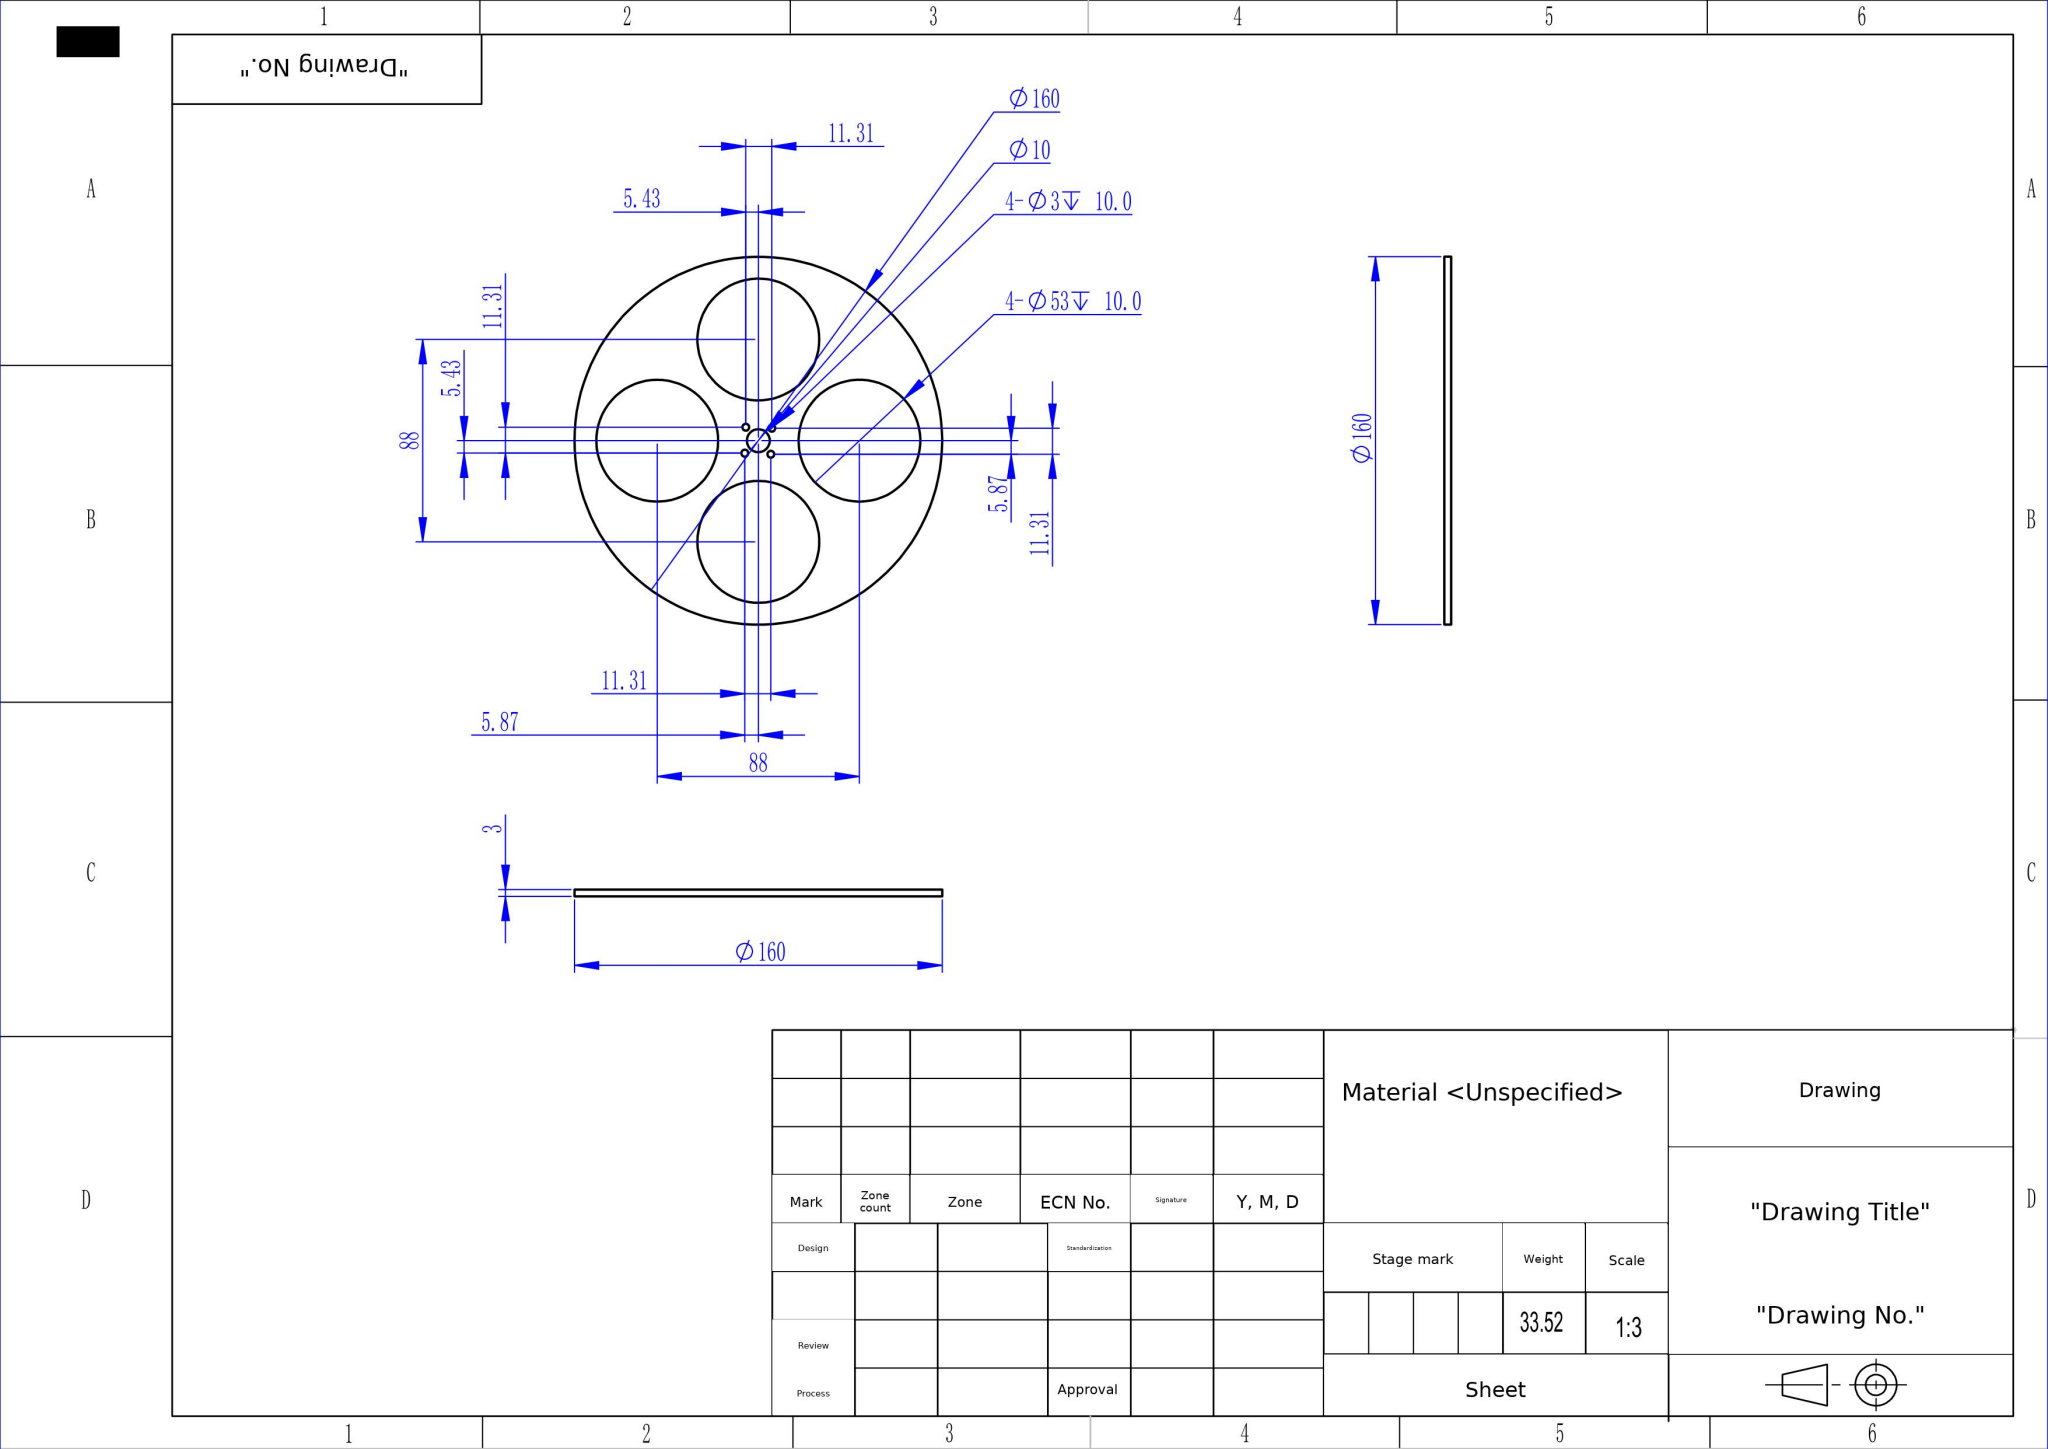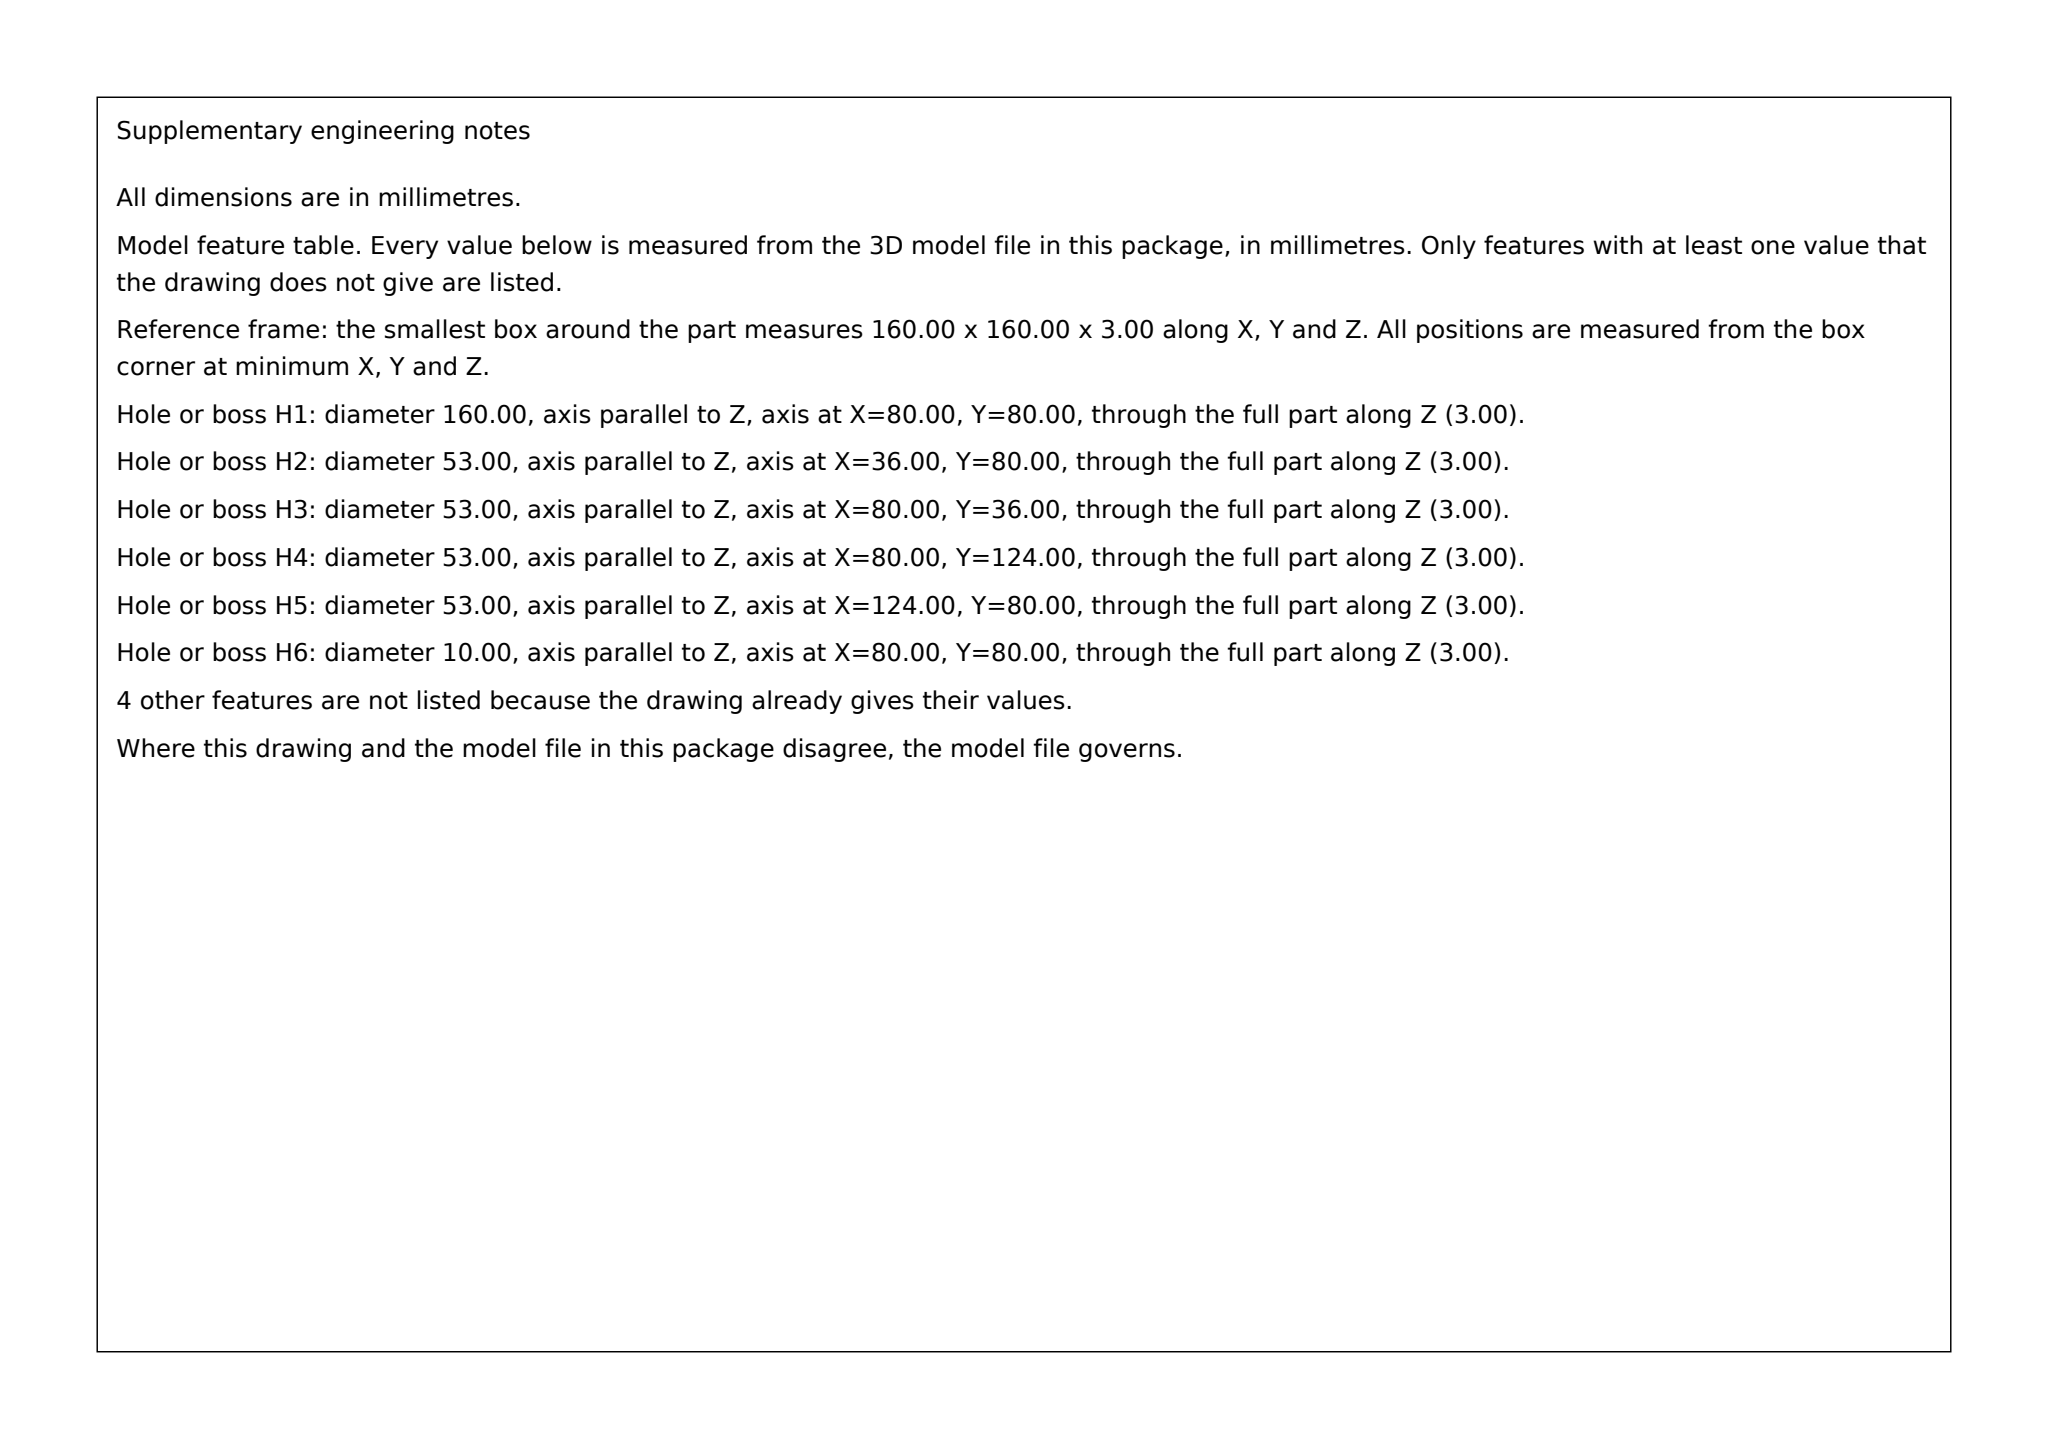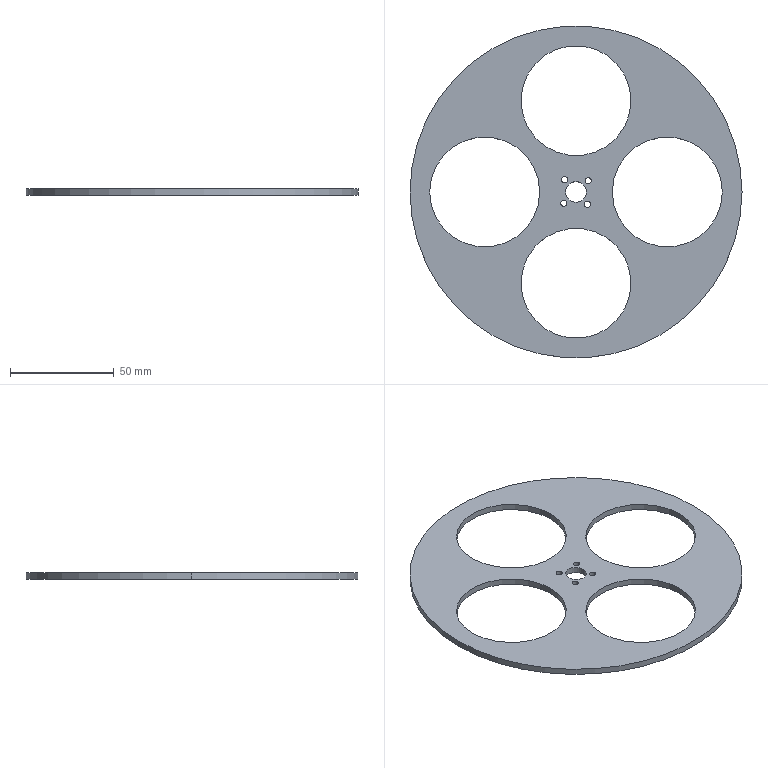Part | SolidWorks | mm | material <Unspecified> | 1 solid | 22 faces | box 160 x 160 x 3 mm | volume 33524 mm3 | cylinder 20 | plane 2 | commonest cylinder face diameters 3 x8 53 x8 10 x2 160 x2
build123d program:
from build123d import *

# Parameters (mm, degrees)
SKETCH1_R           = 80
SKETCH1_R_2         = 5
BOSS_EXTRUDE1_DEPTH = 3
SKETCH4_R           = 26.5
CUT_EXTRUDE2_DEPTH  = 10
CIRPATTERN1_COUNT   = 4
SKETCH5_R           = 1.5
CUT_EXTRUDE3_DEPTH  = 10


with BuildPart() as part:
    # Sketch1 → Boss-Extrude1 (new body)
    with BuildSketch(Plane.XY):
        Circle(SKETCH1_R)
        Circle(SKETCH1_R_2, mode=Mode.SUBTRACT)
    extrude(amount=BOSS_EXTRUDE1_DEPTH)

    # Sketch4 → Cut-Extrude2 (cut)
    with BuildSketch(Plane.XY.offset(3)):
        with Locations((0, 44)):
            Circle(SKETCH4_R)
    cut_extrude2 = extrude(amount=-CUT_EXTRUDE2_DEPTH, mode=Mode.SUBTRACT)

    # CirPattern1: Cut-Extrude2 ×4 about axis
    cirpattern1_axis = Axis((0, 0, 0), (0, 0, 1))
    for i in range(1, CIRPATTERN1_COUNT):
        add(cut_extrude2.rotate(cirpattern1_axis, i * 360 / CIRPATTERN1_COUNT), mode=Mode.SUBTRACT)

    # Sketch5 → Cut-Extrude3 (cut)
    with BuildSketch(Plane.XY.offset(3)):
        with Locations((-5.434, 5.871)):
            Circle(SKETCH5_R)
        with Locations((5.871, 5.434)):
            Circle(SKETCH5_R)
        with Locations((5.434, -5.871)):
            Circle(SKETCH5_R)
        with Locations((-5.871, -5.434)):
            Circle(SKETCH5_R)
    extrude(amount=-CUT_EXTRUDE3_DEPTH, mode=Mode.SUBTRACT)


solid = part.part
STEP:
#1=CARTESIAN_POINT('',(-7.371,-5.434,0.));
#2=VERTEX_POINT('',#1);
#3=CARTESIAN_POINT('',(-4.371,-5.434,0.));
#4=VERTEX_POINT('',#3);
#5=CARTESIAN_POINT('',(-5.871,-5.434,0.));
#6=DIRECTION('',(0.,0.,1.));
#7=DIRECTION('',(1.,0.,0.));
#8=AXIS2_PLACEMENT_3D('',#5,#6,#7);
#9=CIRCLE('',#8,1.5);
#10=EDGE_CURVE('',#2,#4,#9,.T.);
#11=ORIENTED_EDGE('',*,*,#10,.F.);
#12=CARTESIAN_POINT('',(-7.371,-5.434,3.));
#13=VERTEX_POINT('',#12);
#14=CARTESIAN_POINT('',(-7.371,-5.434,-7.));
#15=DIRECTION('',(0.,0.,1.));
#16=VECTOR('',#15,1000.);
#17=LINE('',#14,#16);
#18=EDGE_CURVE('',#2,#13,#17,.T.);
#19=ORIENTED_EDGE('',*,*,#18,.T.);
#20=CARTESIAN_POINT('',(-4.371,-5.434,3.));
#21=VERTEX_POINT('',#20);
#22=CARTESIAN_POINT('',(-5.871,-5.434,3.));
#23=DIRECTION('',(0.,0.,1.));
#24=DIRECTION('',(1.,0.,0.));
#25=AXIS2_PLACEMENT_3D('',#22,#23,#24);
#26=CIRCLE('',#25,1.5);
#27=EDGE_CURVE('',#13,#21,#26,.T.);
#28=ORIENTED_EDGE('',*,*,#27,.T.);
#29=CARTESIAN_POINT('',(-4.371,-5.434,-7.));
#30=DIRECTION('',(0.,0.,1.));
#31=VECTOR('',#30,1000.);
#32=LINE('',#29,#31);
#33=EDGE_CURVE('',#4,#21,#32,.T.);
#34=ORIENTED_EDGE('',*,*,#33,.F.);
#35=EDGE_LOOP('',(#11,#19,#28,#34));
#36=FACE_OUTER_BOUND('',#35,.T.);
#37=CARTESIAN_POINT('',(-5.871,-5.434,-7.));
#38=DIRECTION('',(0.,0.,1.));
#39=DIRECTION('',(1.,0.,0.));
#40=AXIS2_PLACEMENT_3D('',#37,#38,#39);
#41=CYLINDRICAL_SURFACE('',#40,1.5);
#42=ADVANCED_FACE('',(#36),#41,.F.);
#43=CARTESIAN_POINT('',(3.934,-5.871,0.));
#44=VERTEX_POINT('',#43);
#45=CARTESIAN_POINT('',(6.934,-5.871,0.));
#46=VERTEX_POINT('',#45);
#47=CARTESIAN_POINT('',(5.434,-5.871,0.));
#48=DIRECTION('',(0.,0.,1.));
#49=DIRECTION('',(1.,0.,0.));
#50=AXIS2_PLACEMENT_3D('',#47,#48,#49);
#51=CIRCLE('',#50,1.5);
#52=EDGE_CURVE('',#44,#46,#51,.T.);
#53=ORIENTED_EDGE('',*,*,#52,.F.);
#54=CARTESIAN_POINT('',(3.934,-5.871,3.));
#55=VERTEX_POINT('',#54);
#56=CARTESIAN_POINT('',(3.934,-5.871,-7.));
#57=DIRECTION('',(0.,0.,1.));
#58=VECTOR('',#57,1000.);
#59=LINE('',#56,#58);
#60=EDGE_CURVE('',#44,#55,#59,.T.);
#61=ORIENTED_EDGE('',*,*,#60,.T.);
#62=CARTESIAN_POINT('',(6.934,-5.871,3.));
#63=VERTEX_POINT('',#62);
#64=CARTESIAN_POINT('',(5.434,-5.871,3.));
#65=DIRECTION('',(0.,0.,1.));
#66=DIRECTION('',(1.,0.,0.));
#67=AXIS2_PLACEMENT_3D('',#64,#65,#66);
#68=CIRCLE('',#67,1.5);
#69=EDGE_CURVE('',#55,#63,#68,.T.);
#70=ORIENTED_EDGE('',*,*,#69,.T.);
#71=CARTESIAN_POINT('',(6.934,-5.871,-7.));
#72=DIRECTION('',(0.,0.,1.));
#73=VECTOR('',#72,1000.);
#74=LINE('',#71,#73);
#75=EDGE_CURVE('',#46,#63,#74,.T.);
#76=ORIENTED_EDGE('',*,*,#75,.F.);
#77=EDGE_LOOP('',(#53,#61,#70,#76));
#78=FACE_OUTER_BOUND('',#77,.T.);
#79=CARTESIAN_POINT('',(5.434,-5.871,-7.));
#80=DIRECTION('',(0.,0.,1.));
#81=DIRECTION('',(1.,0.,0.));
#82=AXIS2_PLACEMENT_3D('',#79,#80,#81);
#83=CYLINDRICAL_SURFACE('',#82,1.5);
#84=ADVANCED_FACE('',(#78),#83,.F.);
#85=CARTESIAN_POINT('',(4.371,5.434,0.));
#86=VERTEX_POINT('',#85);
#87=CARTESIAN_POINT('',(7.371,5.434,0.));
#88=VERTEX_POINT('',#87);
#89=CARTESIAN_POINT('',(5.871,5.434,0.));
#90=DIRECTION('',(0.,0.,1.));
#91=DIRECTION('',(1.,0.,0.));
#92=AXIS2_PLACEMENT_3D('',#89,#90,#91);
#93=CIRCLE('',#92,1.5);
#94=EDGE_CURVE('',#86,#88,#93,.T.);
#95=ORIENTED_EDGE('',*,*,#94,.F.);
#96=CARTESIAN_POINT('',(4.371,5.434,3.));
#97=VERTEX_POINT('',#96);
#98=CARTESIAN_POINT('',(4.371,5.434,-7.));
#99=DIRECTION('',(0.,0.,1.));
#100=VECTOR('',#99,1000.);
#101=LINE('',#98,#100);
#102=EDGE_CURVE('',#86,#97,#101,.T.);
#103=ORIENTED_EDGE('',*,*,#102,.T.);
#104=CARTESIAN_POINT('',(7.371,5.434,3.));
#105=VERTEX_POINT('',#104);
#106=CARTESIAN_POINT('',(5.871,5.434,3.));
#107=DIRECTION('',(0.,0.,1.));
#108=DIRECTION('',(1.,0.,0.));
#109=AXIS2_PLACEMENT_3D('',#106,#107,#108);
#110=CIRCLE('',#109,1.5);
#111=EDGE_CURVE('',#97,#105,#110,.T.);
#112=ORIENTED_EDGE('',*,*,#111,.T.);
#113=CARTESIAN_POINT('',(7.371,5.434,-7.));
#114=DIRECTION('',(0.,0.,1.));
#115=VECTOR('',#114,1000.);
#116=LINE('',#113,#115);
#117=EDGE_CURVE('',#88,#105,#116,.T.);
#118=ORIENTED_EDGE('',*,*,#117,.F.);
#119=EDGE_LOOP('',(#95,#103,#112,#118));
#120=FACE_OUTER_BOUND('',#119,.T.);
#121=CARTESIAN_POINT('',(5.871,5.434,-7.));
#122=DIRECTION('',(0.,0.,1.));
#123=DIRECTION('',(1.,0.,0.));
#124=AXIS2_PLACEMENT_3D('',#121,#122,#123);
#125=CYLINDRICAL_SURFACE('',#124,1.5);
#126=ADVANCED_FACE('',(#120),#125,.F.);
#127=CARTESIAN_POINT('',(-6.934,5.871,0.));
#128=VERTEX_POINT('',#127);
#129=CARTESIAN_POINT('',(-3.934,5.871,0.));
#130=VERTEX_POINT('',#129);
#131=CARTESIAN_POINT('',(-5.434,5.871,0.));
#132=DIRECTION('',(0.,0.,1.));
#133=DIRECTION('',(1.,0.,0.));
#134=AXIS2_PLACEMENT_3D('',#131,#132,#133);
#135=CIRCLE('',#134,1.5);
#136=EDGE_CURVE('',#128,#130,#135,.T.);
#137=ORIENTED_EDGE('',*,*,#136,.F.);
#138=CARTESIAN_POINT('',(-6.934,5.871,3.));
#139=VERTEX_POINT('',#138);
#140=CARTESIAN_POINT('',(-6.934,5.871,-7.));
#141=DIRECTION('',(0.,0.,1.));
#142=VECTOR('',#141,1000.);
#143=LINE('',#140,#142);
#144=EDGE_CURVE('',#128,#139,#143,.T.);
#145=ORIENTED_EDGE('',*,*,#144,.T.);
#146=CARTESIAN_POINT('',(-3.934,5.871,3.));
#147=VERTEX_POINT('',#146);
#148=CARTESIAN_POINT('',(-5.434,5.871,3.));
#149=DIRECTION('',(0.,0.,1.));
#150=DIRECTION('',(1.,0.,0.));
#151=AXIS2_PLACEMENT_3D('',#148,#149,#150);
#152=CIRCLE('',#151,1.5);
#153=EDGE_CURVE('',#139,#147,#152,.T.);
#154=ORIENTED_EDGE('',*,*,#153,.T.);
#155=CARTESIAN_POINT('',(-3.934,5.871,-7.));
#156=DIRECTION('',(0.,0.,1.));
#157=VECTOR('',#156,1000.);
#158=LINE('',#155,#157);
#159=EDGE_CURVE('',#130,#147,#158,.T.);
#160=ORIENTED_EDGE('',*,*,#159,.F.);
#161=EDGE_LOOP('',(#137,#145,#154,#160));
#162=FACE_OUTER_BOUND('',#161,.T.);
#163=CARTESIAN_POINT('',(-5.434,5.871,-7.));
#164=DIRECTION('',(0.,0.,1.));
#165=DIRECTION('',(1.,0.,0.));
#166=AXIS2_PLACEMENT_3D('',#163,#164,#165);
#167=CYLINDRICAL_SURFACE('',#166,1.5);
#168=ADVANCED_FACE('',(#162),#167,.F.);
#169=CARTESIAN_POINT('',(-26.5,-44.,0.));
#170=VERTEX_POINT('',#169);
#171=CARTESIAN_POINT('',(26.5,-44.,0.));
#172=VERTEX_POINT('',#171);
#173=CARTESIAN_POINT('',(0.,-44.,0.));
#174=DIRECTION('',(0.,0.,1.));
#175=DIRECTION('',(1.,0.,0.));
#176=AXIS2_PLACEMENT_3D('',#173,#174,#175);
#177=CIRCLE('',#176,26.5);
#178=EDGE_CURVE('',#170,#172,#177,.T.);
#179=ORIENTED_EDGE('',*,*,#178,.F.);
#180=CARTESIAN_POINT('',(-26.5,-44.,3.));
#181=VERTEX_POINT('',#180);
#182=CARTESIAN_POINT('',(-26.5,-44.,-7.));
#183=DIRECTION('',(0.,0.,1.));
#184=VECTOR('',#183,1000.);
#185=LINE('',#182,#184);
#186=EDGE_CURVE('',#170,#181,#185,.T.);
#187=ORIENTED_EDGE('',*,*,#186,.T.);
#188=CARTESIAN_POINT('',(26.5,-44.,3.));
#189=VERTEX_POINT('',#188);
#190=CARTESIAN_POINT('',(0.,-44.,3.));
#191=DIRECTION('',(0.,0.,1.));
#192=DIRECTION('',(-1.,0.,0.));
#193=AXIS2_PLACEMENT_3D('',#190,#191,#192);
#194=CIRCLE('',#193,26.5);
#195=EDGE_CURVE('',#181,#189,#194,.T.);
#196=ORIENTED_EDGE('',*,*,#195,.T.);
#197=CARTESIAN_POINT('',(26.5,-44.,-7.));
#198=DIRECTION('',(0.,0.,1.));
#199=VECTOR('',#198,1000.);
#200=LINE('',#197,#199);
#201=EDGE_CURVE('',#172,#189,#200,.T.);
#202=ORIENTED_EDGE('',*,*,#201,.F.);
#203=EDGE_LOOP('',(#179,#187,#196,#202));
#204=FACE_OUTER_BOUND('',#203,.T.);
#205=CARTESIAN_POINT('',(0.,-44.,-7.));
#206=DIRECTION('',(0.,0.,1.));
#207=DIRECTION('',(1.,0.,0.));
#208=AXIS2_PLACEMENT_3D('',#205,#206,#207);
#209=CYLINDRICAL_SURFACE('',#208,26.5);
#210=ADVANCED_FACE('',(#204),#209,.F.);
#211=CARTESIAN_POINT('',(17.5,0.,0.));
#212=VERTEX_POINT('',#211);
#213=CARTESIAN_POINT('',(70.5,0.,0.));
#214=VERTEX_POINT('',#213);
#215=CARTESIAN_POINT('',(44.,0.,0.));
#216=DIRECTION('',(0.,0.,1.));
#217=DIRECTION('',(1.,0.,0.));
#218=AXIS2_PLACEMENT_3D('',#215,#216,#217);
#219=CIRCLE('',#218,26.5);
#220=EDGE_CURVE('',#212,#214,#219,.T.);
#221=ORIENTED_EDGE('',*,*,#220,.F.);
#222=CARTESIAN_POINT('',(17.5,0.,3.));
#223=VERTEX_POINT('',#222);
#224=CARTESIAN_POINT('',(17.5,0.,-7.));
#225=DIRECTION('',(0.,0.,1.));
#226=VECTOR('',#225,1000.);
#227=LINE('',#224,#226);
#228=EDGE_CURVE('',#212,#223,#227,.T.);
#229=ORIENTED_EDGE('',*,*,#228,.T.);
#230=CARTESIAN_POINT('',(70.5,0.,3.));
#231=VERTEX_POINT('',#230);
#232=CARTESIAN_POINT('',(44.,0.,3.));
#233=DIRECTION('',(0.,0.,1.));
#234=DIRECTION('',(0.,-1.,0.));
#235=AXIS2_PLACEMENT_3D('',#232,#233,#234);
#236=CIRCLE('',#235,26.5);
#237=EDGE_CURVE('',#223,#231,#236,.T.);
#238=ORIENTED_EDGE('',*,*,#237,.T.);
#239=CARTESIAN_POINT('',(70.5,0.,-7.));
#240=DIRECTION('',(0.,0.,1.));
#241=VECTOR('',#240,1000.);
#242=LINE('',#239,#241);
#243=EDGE_CURVE('',#214,#231,#242,.T.);
#244=ORIENTED_EDGE('',*,*,#243,.F.);
#245=EDGE_LOOP('',(#221,#229,#238,#244));
#246=FACE_OUTER_BOUND('',#245,.T.);
#247=CARTESIAN_POINT('',(44.,0.,-7.));
#248=DIRECTION('',(0.,0.,1.));
#249=DIRECTION('',(1.,0.,0.));
#250=AXIS2_PLACEMENT_3D('',#247,#248,#249);
#251=CYLINDRICAL_SURFACE('',#250,26.5);
#252=ADVANCED_FACE('',(#246),#251,.F.);
#253=CARTESIAN_POINT('',(-70.5,-0.,0.));
#254=VERTEX_POINT('',#253);
#255=CARTESIAN_POINT('',(-17.5,-0.,0.));
#256=VERTEX_POINT('',#255);
#257=CARTESIAN_POINT('',(-44.,-0.,0.));
#258=DIRECTION('',(0.,0.,1.));
#259=DIRECTION('',(1.,0.,0.));
#260=AXIS2_PLACEMENT_3D('',#257,#258,#259);
#261=CIRCLE('',#260,26.5);
#262=EDGE_CURVE('',#254,#256,#261,.T.);
#263=ORIENTED_EDGE('',*,*,#262,.F.);
#264=CARTESIAN_POINT('',(-70.5,-0.,3.));
#265=VERTEX_POINT('',#264);
#266=CARTESIAN_POINT('',(-70.5,-0.,-7.));
#267=DIRECTION('',(0.,0.,1.));
#268=VECTOR('',#267,1000.);
#269=LINE('',#266,#268);
#270=EDGE_CURVE('',#254,#265,#269,.T.);
#271=ORIENTED_EDGE('',*,*,#270,.T.);
#272=CARTESIAN_POINT('',(-17.5,-0.,3.));
#273=VERTEX_POINT('',#272);
#274=CARTESIAN_POINT('',(-44.,-0.,3.));
#275=DIRECTION('',(0.,0.,1.));
#276=DIRECTION('',(-0.,1.,0.));
#277=AXIS2_PLACEMENT_3D('',#274,#275,#276);
#278=CIRCLE('',#277,26.5);
#279=EDGE_CURVE('',#265,#273,#278,.T.);
#280=ORIENTED_EDGE('',*,*,#279,.T.);
#281=CARTESIAN_POINT('',(-17.5,-0.,-7.));
#282=DIRECTION('',(0.,0.,1.));
#283=VECTOR('',#282,1000.);
#284=LINE('',#281,#283);
#285=EDGE_CURVE('',#256,#273,#284,.T.);
#286=ORIENTED_EDGE('',*,*,#285,.F.);
#287=EDGE_LOOP('',(#263,#271,#280,#286));
#288=FACE_OUTER_BOUND('',#287,.T.);
#289=CARTESIAN_POINT('',(-44.,-0.,-7.));
#290=DIRECTION('',(0.,0.,1.));
#291=DIRECTION('',(1.,0.,0.));
#292=AXIS2_PLACEMENT_3D('',#289,#290,#291);
#293=CYLINDRICAL_SURFACE('',#292,26.5);
#294=ADVANCED_FACE('',(#288),#293,.F.);
#295=CARTESIAN_POINT('',(-26.5,44.,0.));
#296=VERTEX_POINT('',#295);
#297=CARTESIAN_POINT('',(26.5,44.,0.));
#298=VERTEX_POINT('',#297);
#299=CARTESIAN_POINT('',(0.,44.,0.));
#300=DIRECTION('',(0.,0.,1.));
#301=DIRECTION('',(1.,0.,0.));
#302=AXIS2_PLACEMENT_3D('',#299,#300,#301);
#303=CIRCLE('',#302,26.5);
#304=EDGE_CURVE('',#296,#298,#303,.T.);
#305=ORIENTED_EDGE('',*,*,#304,.F.);
#306=CARTESIAN_POINT('',(-26.5,44.,3.));
#307=VERTEX_POINT('',#306);
#308=CARTESIAN_POINT('',(-26.5,44.,-7.));
#309=DIRECTION('',(0.,0.,1.));
#310=VECTOR('',#309,1000.);
#311=LINE('',#308,#310);
#312=EDGE_CURVE('',#296,#307,#311,.T.);
#313=ORIENTED_EDGE('',*,*,#312,.T.);
#314=CARTESIAN_POINT('',(26.5,44.,3.));
#315=VERTEX_POINT('',#314);
#316=CARTESIAN_POINT('',(0.,44.,3.));
#317=DIRECTION('',(0.,0.,1.));
#318=DIRECTION('',(1.,0.,0.));
#319=AXIS2_PLACEMENT_3D('',#316,#317,#318);
#320=CIRCLE('',#319,26.5);
#321=EDGE_CURVE('',#307,#315,#320,.T.);
#322=ORIENTED_EDGE('',*,*,#321,.T.);
#323=CARTESIAN_POINT('',(26.5,44.,-7.));
#324=DIRECTION('',(0.,0.,1.));
#325=VECTOR('',#324,1000.);
#326=LINE('',#323,#325);
#327=EDGE_CURVE('',#298,#315,#326,.T.);
#328=ORIENTED_EDGE('',*,*,#327,.F.);
#329=EDGE_LOOP('',(#305,#313,#322,#328));
#330=FACE_OUTER_BOUND('',#329,.T.);
#331=CARTESIAN_POINT('',(0.,44.,-7.));
#332=DIRECTION('',(0.,0.,1.));
#333=DIRECTION('',(1.,0.,0.));
#334=AXIS2_PLACEMENT_3D('',#331,#332,#333);
#335=CYLINDRICAL_SURFACE('',#334,26.5);
#336=ADVANCED_FACE('',(#330),#335,.F.);
#337=CARTESIAN_POINT('',(-5.,0.,3.));
#338=VERTEX_POINT('',#337);
#339=CARTESIAN_POINT('',(5.,0.,3.));
#340=VERTEX_POINT('',#339);
#341=CARTESIAN_POINT('',(0.,0.,3.));
#342=DIRECTION('',(0.,0.,1.));
#343=DIRECTION('',(1.,0.,0.));
#344=AXIS2_PLACEMENT_3D('',#341,#342,#343);
#345=CIRCLE('',#344,5.);
#346=EDGE_CURVE('',#338,#340,#345,.T.);
#347=ORIENTED_EDGE('',*,*,#346,.T.);
#348=CARTESIAN_POINT('',(5.,0.,0.));
#349=VERTEX_POINT('',#348);
#350=CARTESIAN_POINT('',(5.,0.,3.));
#351=DIRECTION('',(0.,0.,-1.));
#352=VECTOR('',#351,1000.);
#353=LINE('',#350,#352);
#354=EDGE_CURVE('',#340,#349,#353,.T.);
#355=ORIENTED_EDGE('',*,*,#354,.T.);
#356=CARTESIAN_POINT('',(-5.,0.,0.));
#357=VERTEX_POINT('',#356);
#358=CARTESIAN_POINT('',(0.,0.,0.));
#359=DIRECTION('',(0.,0.,1.));
#360=DIRECTION('',(1.,0.,0.));
#361=AXIS2_PLACEMENT_3D('',#358,#359,#360);
#362=CIRCLE('',#361,5.);
#363=EDGE_CURVE('',#357,#349,#362,.T.);
#364=ORIENTED_EDGE('',*,*,#363,.F.);
#365=CARTESIAN_POINT('',(-5.,0.,3.));
#366=DIRECTION('',(0.,0.,-1.));
#367=VECTOR('',#366,1000.);
#368=LINE('',#365,#367);
#369=EDGE_CURVE('',#338,#357,#368,.T.);
#370=ORIENTED_EDGE('',*,*,#369,.F.);
#371=EDGE_LOOP('',(#347,#355,#364,#370));
#372=FACE_OUTER_BOUND('',#371,.T.);
#373=CARTESIAN_POINT('',(0.,0.,3.));
#374=DIRECTION('',(0.,0.,-1.));
#375=DIRECTION('',(-1.,0.,0.));
#376=AXIS2_PLACEMENT_3D('',#373,#374,#375);
#377=CYLINDRICAL_SURFACE('',#376,5.);
#378=ADVANCED_FACE('',(#372),#377,.F.);
#379=CARTESIAN_POINT('',(80.,0.,3.));
#380=VERTEX_POINT('',#379);
#381=CARTESIAN_POINT('',(-80.,0.,3.));
#382=VERTEX_POINT('',#381);
#383=CARTESIAN_POINT('',(0.,0.,3.));
#384=DIRECTION('',(0.,0.,1.));
#385=DIRECTION('',(1.,0.,0.));
#386=AXIS2_PLACEMENT_3D('',#383,#384,#385);
#387=CIRCLE('',#386,80.);
#388=EDGE_CURVE('',#380,#382,#387,.T.);
#389=ORIENTED_EDGE('',*,*,#388,.F.);
#390=CARTESIAN_POINT('',(80.,0.,0.));
#391=VERTEX_POINT('',#390);
#392=CARTESIAN_POINT('',(80.,0.,3.));
#393=DIRECTION('',(0.,0.,-1.));
#394=VECTOR('',#393,1000.);
#395=LINE('',#392,#394);
#396=EDGE_CURVE('',#380,#391,#395,.T.);
#397=ORIENTED_EDGE('',*,*,#396,.T.);
#398=CARTESIAN_POINT('',(-80.,0.,0.));
#399=VERTEX_POINT('',#398);
#400=CARTESIAN_POINT('',(0.,0.,0.));
#401=DIRECTION('',(0.,0.,1.));
#402=DIRECTION('',(1.,0.,0.));
#403=AXIS2_PLACEMENT_3D('',#400,#401,#402);
#404=CIRCLE('',#403,80.);
#405=EDGE_CURVE('',#391,#399,#404,.T.);
#406=ORIENTED_EDGE('',*,*,#405,.T.);
#407=CARTESIAN_POINT('',(-80.,0.,3.));
#408=DIRECTION('',(0.,0.,-1.));
#409=VECTOR('',#408,1000.);
#410=LINE('',#407,#409);
#411=EDGE_CURVE('',#382,#399,#410,.T.);
#412=ORIENTED_EDGE('',*,*,#411,.F.);
#413=EDGE_LOOP('',(#389,#397,#406,#412));
#414=FACE_OUTER_BOUND('',#413,.T.);
#415=CARTESIAN_POINT('',(0.,0.,3.));
#416=DIRECTION('',(0.,0.,-1.));
#417=DIRECTION('',(-1.,0.,0.));
#418=AXIS2_PLACEMENT_3D('',#415,#416,#417);
#419=CYLINDRICAL_SURFACE('',#418,80.);
#420=ADVANCED_FACE('',(#414),#419,.T.);
#421=CARTESIAN_POINT('',(-5.871,-5.434,3.));
#422=DIRECTION('',(0.,0.,1.));
#423=DIRECTION('',(1.,0.,0.));
#424=AXIS2_PLACEMENT_3D('',#421,#422,#423);
#425=CIRCLE('',#424,1.5);
#426=EDGE_CURVE('',#21,#13,#425,.T.);
#427=ORIENTED_EDGE('',*,*,#426,.F.);
#428=ORIENTED_EDGE('',*,*,#27,.F.);
#429=EDGE_LOOP('',(#427,#428));
#430=FACE_BOUND('',#429,.T.);
#431=CARTESIAN_POINT('',(5.434,-5.871,3.));
#432=DIRECTION('',(0.,0.,1.));
#433=DIRECTION('',(1.,0.,0.));
#434=AXIS2_PLACEMENT_3D('',#431,#432,#433);
#435=CIRCLE('',#434,1.5);
#436=EDGE_CURVE('',#63,#55,#435,.T.);
#437=ORIENTED_EDGE('',*,*,#436,.F.);
#438=ORIENTED_EDGE('',*,*,#69,.F.);
#439=EDGE_LOOP('',(#437,#438));
#440=FACE_BOUND('',#439,.T.);
#441=CARTESIAN_POINT('',(5.871,5.434,3.));
#442=DIRECTION('',(0.,0.,1.));
#443=DIRECTION('',(1.,0.,0.));
#444=AXIS2_PLACEMENT_3D('',#441,#442,#443);
#445=CIRCLE('',#444,1.5);
#446=EDGE_CURVE('',#105,#97,#445,.T.);
#447=ORIENTED_EDGE('',*,*,#446,.F.);
#448=ORIENTED_EDGE('',*,*,#111,.F.);
#449=EDGE_LOOP('',(#447,#448));
#450=FACE_BOUND('',#449,.T.);
#451=CARTESIAN_POINT('',(-5.434,5.871,3.));
#452=DIRECTION('',(0.,0.,1.));
#453=DIRECTION('',(1.,0.,0.));
#454=AXIS2_PLACEMENT_3D('',#451,#452,#453);
#455=CIRCLE('',#454,1.5);
#456=EDGE_CURVE('',#147,#139,#455,.T.);
#457=ORIENTED_EDGE('',*,*,#456,.F.);
#458=ORIENTED_EDGE('',*,*,#153,.F.);
#459=EDGE_LOOP('',(#457,#458));
#460=FACE_BOUND('',#459,.T.);
#461=CARTESIAN_POINT('',(0.,-44.,3.));
#462=DIRECTION('',(0.,0.,1.));
#463=DIRECTION('',(-1.,0.,0.));
#464=AXIS2_PLACEMENT_3D('',#461,#462,#463);
#465=CIRCLE('',#464,26.5);
#466=EDGE_CURVE('',#189,#181,#465,.T.);
#467=ORIENTED_EDGE('',*,*,#466,.F.);
#468=ORIENTED_EDGE('',*,*,#195,.F.);
#469=EDGE_LOOP('',(#467,#468));
#470=FACE_BOUND('',#469,.T.);
#471=CARTESIAN_POINT('',(44.,0.,3.));
#472=DIRECTION('',(0.,0.,1.));
#473=DIRECTION('',(0.,-1.,0.));
#474=AXIS2_PLACEMENT_3D('',#471,#472,#473);
#475=CIRCLE('',#474,26.5);
#476=EDGE_CURVE('',#231,#223,#475,.T.);
#477=ORIENTED_EDGE('',*,*,#476,.F.);
#478=ORIENTED_EDGE('',*,*,#237,.F.);
#479=EDGE_LOOP('',(#477,#478));
#480=FACE_BOUND('',#479,.T.);
#481=CARTESIAN_POINT('',(-44.,-0.,3.));
#482=DIRECTION('',(0.,0.,1.));
#483=DIRECTION('',(-0.,1.,0.));
#484=AXIS2_PLACEMENT_3D('',#481,#482,#483);
#485=CIRCLE('',#484,26.5);
#486=EDGE_CURVE('',#273,#265,#485,.T.);
#487=ORIENTED_EDGE('',*,*,#486,.F.);
#488=ORIENTED_EDGE('',*,*,#279,.F.);
#489=EDGE_LOOP('',(#487,#488));
#490=FACE_BOUND('',#489,.T.);
#491=CARTESIAN_POINT('',(0.,44.,3.));
#492=DIRECTION('',(0.,0.,1.));
#493=DIRECTION('',(1.,0.,0.));
#494=AXIS2_PLACEMENT_3D('',#491,#492,#493);
#495=CIRCLE('',#494,26.5);
#496=EDGE_CURVE('',#315,#307,#495,.T.);
#497=ORIENTED_EDGE('',*,*,#496,.F.);
#498=ORIENTED_EDGE('',*,*,#321,.F.);
#499=EDGE_LOOP('',(#497,#498));
#500=FACE_BOUND('',#499,.T.);
#501=CARTESIAN_POINT('',(0.,0.,3.));
#502=DIRECTION('',(0.,0.,1.));
#503=DIRECTION('',(1.,0.,0.));
#504=AXIS2_PLACEMENT_3D('',#501,#502,#503);
#505=CIRCLE('',#504,80.);
#506=EDGE_CURVE('',#382,#380,#505,.T.);
#507=ORIENTED_EDGE('',*,*,#506,.T.);
#508=ORIENTED_EDGE('',*,*,#388,.T.);
#509=EDGE_LOOP('',(#507,#508));
#510=FACE_OUTER_BOUND('',#509,.T.);
#511=ORIENTED_EDGE('',*,*,#346,.F.);
#512=CARTESIAN_POINT('',(0.,0.,3.));
#513=DIRECTION('',(0.,0.,1.));
#514=DIRECTION('',(1.,0.,0.));
#515=AXIS2_PLACEMENT_3D('',#512,#513,#514);
#516=CIRCLE('',#515,5.);
#517=EDGE_CURVE('',#340,#338,#516,.T.);
#518=ORIENTED_EDGE('',*,*,#517,.F.);
#519=EDGE_LOOP('',(#511,#518));
#520=FACE_BOUND('',#519,.T.);
#521=CARTESIAN_POINT('',(0.,0.,3.));
#522=DIRECTION('',(0.,0.,1.));
#523=DIRECTION('',(1.,0.,0.));
#524=AXIS2_PLACEMENT_3D('',#521,#522,#523);
#525=PLANE('',#524);
#526=ADVANCED_FACE('',(#430,#440,#450,#460,#470,#480,#490,#500,#510,#520),#525,.T.);
#527=CARTESIAN_POINT('',(-5.871,-5.434,0.));
#528=DIRECTION('',(0.,0.,1.));
#529=DIRECTION('',(1.,0.,0.));
#530=AXIS2_PLACEMENT_3D('',#527,#528,#529);
#531=CIRCLE('',#530,1.5);
#532=EDGE_CURVE('',#4,#2,#531,.T.);
#533=ORIENTED_EDGE('',*,*,#532,.T.);
#534=ORIENTED_EDGE('',*,*,#10,.T.);
#535=EDGE_LOOP('',(#533,#534));
#536=FACE_BOUND('',#535,.T.);
#537=CARTESIAN_POINT('',(5.434,-5.871,0.));
#538=DIRECTION('',(0.,0.,1.));
#539=DIRECTION('',(1.,0.,0.));
#540=AXIS2_PLACEMENT_3D('',#537,#538,#539);
#541=CIRCLE('',#540,1.5);
#542=EDGE_CURVE('',#46,#44,#541,.T.);
#543=ORIENTED_EDGE('',*,*,#542,.T.);
#544=ORIENTED_EDGE('',*,*,#52,.T.);
#545=EDGE_LOOP('',(#543,#544));
#546=FACE_BOUND('',#545,.T.);
#547=CARTESIAN_POINT('',(5.871,5.434,0.));
#548=DIRECTION('',(0.,0.,1.));
#549=DIRECTION('',(1.,0.,0.));
#550=AXIS2_PLACEMENT_3D('',#547,#548,#549);
#551=CIRCLE('',#550,1.5);
#552=EDGE_CURVE('',#88,#86,#551,.T.);
#553=ORIENTED_EDGE('',*,*,#552,.T.);
#554=ORIENTED_EDGE('',*,*,#94,.T.);
#555=EDGE_LOOP('',(#553,#554));
#556=FACE_BOUND('',#555,.T.);
#557=CARTESIAN_POINT('',(-5.434,5.871,0.));
#558=DIRECTION('',(0.,0.,1.));
#559=DIRECTION('',(1.,0.,0.));
#560=AXIS2_PLACEMENT_3D('',#557,#558,#559);
#561=CIRCLE('',#560,1.5);
#562=EDGE_CURVE('',#130,#128,#561,.T.);
#563=ORIENTED_EDGE('',*,*,#562,.T.);
#564=ORIENTED_EDGE('',*,*,#136,.T.);
#565=EDGE_LOOP('',(#563,#564));
#566=FACE_BOUND('',#565,.T.);
#567=CARTESIAN_POINT('',(0.,-44.,0.));
#568=DIRECTION('',(0.,0.,1.));
#569=DIRECTION('',(1.,0.,0.));
#570=AXIS2_PLACEMENT_3D('',#567,#568,#569);
#571=CIRCLE('',#570,26.5);
#572=EDGE_CURVE('',#172,#170,#571,.T.);
#573=ORIENTED_EDGE('',*,*,#572,.T.);
#574=ORIENTED_EDGE('',*,*,#178,.T.);
#575=EDGE_LOOP('',(#573,#574));
#576=FACE_BOUND('',#575,.T.);
#577=CARTESIAN_POINT('',(44.,0.,0.));
#578=DIRECTION('',(0.,0.,1.));
#579=DIRECTION('',(1.,0.,0.));
#580=AXIS2_PLACEMENT_3D('',#577,#578,#579);
#581=CIRCLE('',#580,26.5);
#582=EDGE_CURVE('',#214,#212,#581,.T.);
#583=ORIENTED_EDGE('',*,*,#582,.T.);
#584=ORIENTED_EDGE('',*,*,#220,.T.);
#585=EDGE_LOOP('',(#583,#584));
#586=FACE_BOUND('',#585,.T.);
#587=CARTESIAN_POINT('',(-44.,-0.,0.));
#588=DIRECTION('',(0.,0.,1.));
#589=DIRECTION('',(1.,0.,0.));
#590=AXIS2_PLACEMENT_3D('',#587,#588,#589);
#591=CIRCLE('',#590,26.5);
#592=EDGE_CURVE('',#256,#254,#591,.T.);
#593=ORIENTED_EDGE('',*,*,#592,.T.);
#594=ORIENTED_EDGE('',*,*,#262,.T.);
#595=EDGE_LOOP('',(#593,#594));
#596=FACE_BOUND('',#595,.T.);
#597=CARTESIAN_POINT('',(0.,44.,0.));
#598=DIRECTION('',(0.,0.,1.));
#599=DIRECTION('',(1.,0.,0.));
#600=AXIS2_PLACEMENT_3D('',#597,#598,#599);
#601=CIRCLE('',#600,26.5);
#602=EDGE_CURVE('',#298,#296,#601,.T.);
#603=ORIENTED_EDGE('',*,*,#602,.T.);
#604=ORIENTED_EDGE('',*,*,#304,.T.);
#605=EDGE_LOOP('',(#603,#604));
#606=FACE_BOUND('',#605,.T.);
#607=CARTESIAN_POINT('',(0.,0.,0.));
#608=DIRECTION('',(0.,0.,1.));
#609=DIRECTION('',(1.,0.,0.));
#610=AXIS2_PLACEMENT_3D('',#607,#608,#609);
#611=CIRCLE('',#610,80.);
#612=EDGE_CURVE('',#399,#391,#611,.T.);
#613=ORIENTED_EDGE('',*,*,#612,.F.);
#614=ORIENTED_EDGE('',*,*,#405,.F.);
#615=EDGE_LOOP('',(#613,#614));
#616=FACE_OUTER_BOUND('',#615,.T.);
#617=ORIENTED_EDGE('',*,*,#363,.T.);
#618=CARTESIAN_POINT('',(0.,0.,0.));
#619=DIRECTION('',(0.,0.,1.));
#620=DIRECTION('',(1.,0.,0.));
#621=AXIS2_PLACEMENT_3D('',#618,#619,#620);
#622=CIRCLE('',#621,5.);
#623=EDGE_CURVE('',#349,#357,#622,.T.);
#624=ORIENTED_EDGE('',*,*,#623,.T.);
#625=EDGE_LOOP('',(#617,#624));
#626=FACE_BOUND('',#625,.T.);
#627=CARTESIAN_POINT('',(0.,0.,0.));
#628=DIRECTION('',(0.,0.,1.));
#629=DIRECTION('',(1.,0.,0.));
#630=AXIS2_PLACEMENT_3D('',#627,#628,#629);
#631=PLANE('',#630);
#632=ADVANCED_FACE('',(#536,#546,#556,#566,#576,#586,#596,#606,#616,#626),#631,.F.);
#633=ORIENTED_EDGE('',*,*,#396,.F.);
#634=ORIENTED_EDGE('',*,*,#506,.F.);
#635=ORIENTED_EDGE('',*,*,#411,.T.);
#636=ORIENTED_EDGE('',*,*,#612,.T.);
#637=EDGE_LOOP('',(#633,#634,#635,#636));
#638=FACE_OUTER_BOUND('',#637,.T.);
#639=CARTESIAN_POINT('',(0.,0.,3.));
#640=DIRECTION('',(0.,0.,-1.));
#641=DIRECTION('',(-1.,0.,0.));
#642=AXIS2_PLACEMENT_3D('',#639,#640,#641);
#643=CYLINDRICAL_SURFACE('',#642,80.);
#644=ADVANCED_FACE('',(#638),#643,.T.);
#645=ORIENTED_EDGE('',*,*,#354,.F.);
#646=ORIENTED_EDGE('',*,*,#517,.T.);
#647=ORIENTED_EDGE('',*,*,#369,.T.);
#648=ORIENTED_EDGE('',*,*,#623,.F.);
#649=EDGE_LOOP('',(#645,#646,#647,#648));
#650=FACE_OUTER_BOUND('',#649,.T.);
#651=CARTESIAN_POINT('',(0.,0.,3.));
#652=DIRECTION('',(0.,0.,-1.));
#653=DIRECTION('',(-1.,0.,0.));
#654=AXIS2_PLACEMENT_3D('',#651,#652,#653);
#655=CYLINDRICAL_SURFACE('',#654,5.);
#656=ADVANCED_FACE('',(#650),#655,.F.);
#657=ORIENTED_EDGE('',*,*,#312,.F.);
#658=ORIENTED_EDGE('',*,*,#602,.F.);
#659=ORIENTED_EDGE('',*,*,#327,.T.);
#660=ORIENTED_EDGE('',*,*,#496,.T.);
#661=EDGE_LOOP('',(#657,#658,#659,#660));
#662=FACE_OUTER_BOUND('',#661,.T.);
#663=CARTESIAN_POINT('',(0.,44.,-7.));
#664=DIRECTION('',(0.,0.,1.));
#665=DIRECTION('',(1.,0.,0.));
#666=AXIS2_PLACEMENT_3D('',#663,#664,#665);
#667=CYLINDRICAL_SURFACE('',#666,26.5);
#668=ADVANCED_FACE('',(#662),#667,.F.);
#669=ORIENTED_EDGE('',*,*,#270,.F.);
#670=ORIENTED_EDGE('',*,*,#592,.F.);
#671=ORIENTED_EDGE('',*,*,#285,.T.);
#672=ORIENTED_EDGE('',*,*,#486,.T.);
#673=EDGE_LOOP('',(#669,#670,#671,#672));
#674=FACE_OUTER_BOUND('',#673,.T.);
#675=CARTESIAN_POINT('',(-44.,-0.,-7.));
#676=DIRECTION('',(0.,0.,1.));
#677=DIRECTION('',(1.,0.,0.));
#678=AXIS2_PLACEMENT_3D('',#675,#676,#677);
#679=CYLINDRICAL_SURFACE('',#678,26.5);
#680=ADVANCED_FACE('',(#674),#679,.F.);
#681=ORIENTED_EDGE('',*,*,#228,.F.);
#682=ORIENTED_EDGE('',*,*,#582,.F.);
#683=ORIENTED_EDGE('',*,*,#243,.T.);
#684=ORIENTED_EDGE('',*,*,#476,.T.);
#685=EDGE_LOOP('',(#681,#682,#683,#684));
#686=FACE_OUTER_BOUND('',#685,.T.);
#687=CARTESIAN_POINT('',(44.,0.,-7.));
#688=DIRECTION('',(0.,0.,1.));
#689=DIRECTION('',(1.,0.,0.));
#690=AXIS2_PLACEMENT_3D('',#687,#688,#689);
#691=CYLINDRICAL_SURFACE('',#690,26.5);
#692=ADVANCED_FACE('',(#686),#691,.F.);
#693=ORIENTED_EDGE('',*,*,#186,.F.);
#694=ORIENTED_EDGE('',*,*,#572,.F.);
#695=ORIENTED_EDGE('',*,*,#201,.T.);
#696=ORIENTED_EDGE('',*,*,#466,.T.);
#697=EDGE_LOOP('',(#693,#694,#695,#696));
#698=FACE_OUTER_BOUND('',#697,.T.);
#699=CARTESIAN_POINT('',(0.,-44.,-7.));
#700=DIRECTION('',(0.,0.,1.));
#701=DIRECTION('',(1.,0.,0.));
#702=AXIS2_PLACEMENT_3D('',#699,#700,#701);
#703=CYLINDRICAL_SURFACE('',#702,26.5);
#704=ADVANCED_FACE('',(#698),#703,.F.);
#705=ORIENTED_EDGE('',*,*,#144,.F.);
#706=ORIENTED_EDGE('',*,*,#562,.F.);
#707=ORIENTED_EDGE('',*,*,#159,.T.);
#708=ORIENTED_EDGE('',*,*,#456,.T.);
#709=EDGE_LOOP('',(#705,#706,#707,#708));
#710=FACE_OUTER_BOUND('',#709,.T.);
#711=CARTESIAN_POINT('',(-5.434,5.871,-7.));
#712=DIRECTION('',(0.,0.,1.));
#713=DIRECTION('',(1.,0.,0.));
#714=AXIS2_PLACEMENT_3D('',#711,#712,#713);
#715=CYLINDRICAL_SURFACE('',#714,1.5);
#716=ADVANCED_FACE('',(#710),#715,.F.);
#717=ORIENTED_EDGE('',*,*,#102,.F.);
#718=ORIENTED_EDGE('',*,*,#552,.F.);
#719=ORIENTED_EDGE('',*,*,#117,.T.);
#720=ORIENTED_EDGE('',*,*,#446,.T.);
#721=EDGE_LOOP('',(#717,#718,#719,#720));
#722=FACE_OUTER_BOUND('',#721,.T.);
#723=CARTESIAN_POINT('',(5.871,5.434,-7.));
#724=DIRECTION('',(0.,0.,1.));
#725=DIRECTION('',(1.,0.,0.));
#726=AXIS2_PLACEMENT_3D('',#723,#724,#725);
#727=CYLINDRICAL_SURFACE('',#726,1.5);
#728=ADVANCED_FACE('',(#722),#727,.F.);
#729=ORIENTED_EDGE('',*,*,#60,.F.);
#730=ORIENTED_EDGE('',*,*,#542,.F.);
#731=ORIENTED_EDGE('',*,*,#75,.T.);
#732=ORIENTED_EDGE('',*,*,#436,.T.);
#733=EDGE_LOOP('',(#729,#730,#731,#732));
#734=FACE_OUTER_BOUND('',#733,.T.);
#735=CARTESIAN_POINT('',(5.434,-5.871,-7.));
#736=DIRECTION('',(0.,0.,1.));
#737=DIRECTION('',(1.,0.,0.));
#738=AXIS2_PLACEMENT_3D('',#735,#736,#737);
#739=CYLINDRICAL_SURFACE('',#738,1.5);
#740=ADVANCED_FACE('',(#734),#739,.F.);
#741=ORIENTED_EDGE('',*,*,#18,.F.);
#742=ORIENTED_EDGE('',*,*,#532,.F.);
#743=ORIENTED_EDGE('',*,*,#33,.T.);
#744=ORIENTED_EDGE('',*,*,#426,.T.);
#745=EDGE_LOOP('',(#741,#742,#743,#744));
#746=FACE_OUTER_BOUND('',#745,.T.);
#747=CARTESIAN_POINT('',(-5.871,-5.434,-7.));
#748=DIRECTION('',(0.,0.,1.));
#749=DIRECTION('',(1.,0.,0.));
#750=AXIS2_PLACEMENT_3D('',#747,#748,#749);
#751=CYLINDRICAL_SURFACE('',#750,1.5);
#752=ADVANCED_FACE('',(#746),#751,.F.);
#753=CLOSED_SHELL('',(#42,#84,#126,#168,#210,#252,#294,#336,#378,#420,#526,#632,#644,#656,#668,#680,#692,#704,#716,#728,#740,#752));
#754=MANIFOLD_SOLID_BREP('',#753);
#755=CARTESIAN_POINT('',(0.,0.,0.));
#756=DIRECTION('',(0.,0.,1.));
#757=DIRECTION('',(1.,0.,0.));
#758=AXIS2_PLACEMENT_3D('',#755,#756,#757);
#759=(LENGTH_UNIT()NAMED_UNIT(*)SI_UNIT(.MILLI.,.METRE.));
#760=UNCERTAINTY_MEASURE_WITH_UNIT(LENGTH_MEASURE(0.00001),#759,'','');
#761=(NAMED_UNIT(*)PLANE_ANGLE_UNIT()SI_UNIT($,.RADIAN.));
#762=(NAMED_UNIT(*)SI_UNIT($,.STERADIAN.)SOLID_ANGLE_UNIT());
#763=(GEOMETRIC_REPRESENTATION_CONTEXT(3)GLOBAL_UNCERTAINTY_ASSIGNED_CONTEXT((#760))GLOBAL_UNIT_ASSIGNED_CONTEXT((#759,#761,#762))REPRESENTATION_CONTEXT('',''));
#764=ADVANCED_BREP_SHAPE_REPRESENTATION('',(#754,#758),#763);